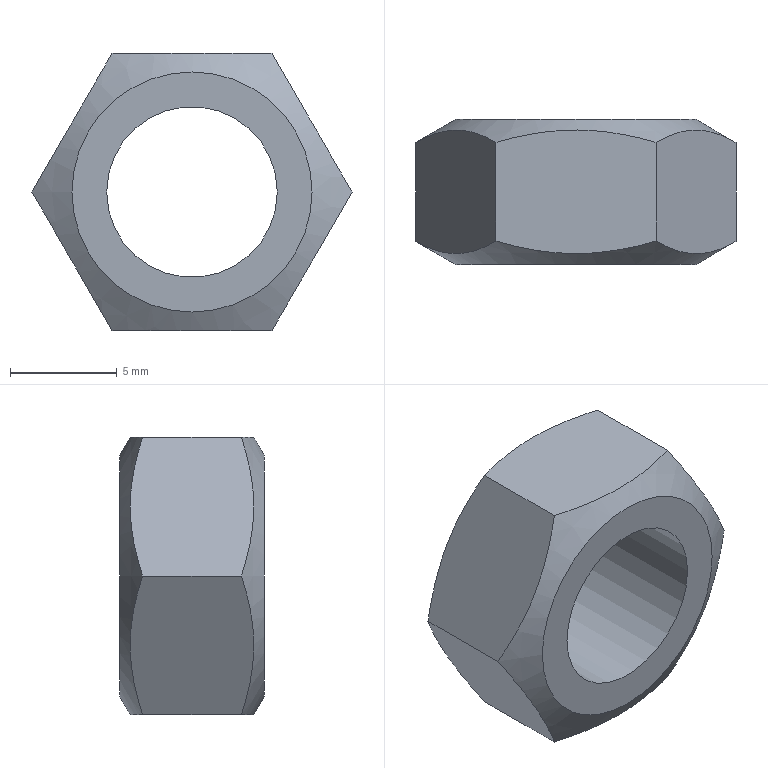Component | NX | NUT | 1 solid | 11 faces | volume 618 mm3 | plane 8 | cone 2 | cylinder 1 | commonest cylinder face diameters 8 x1